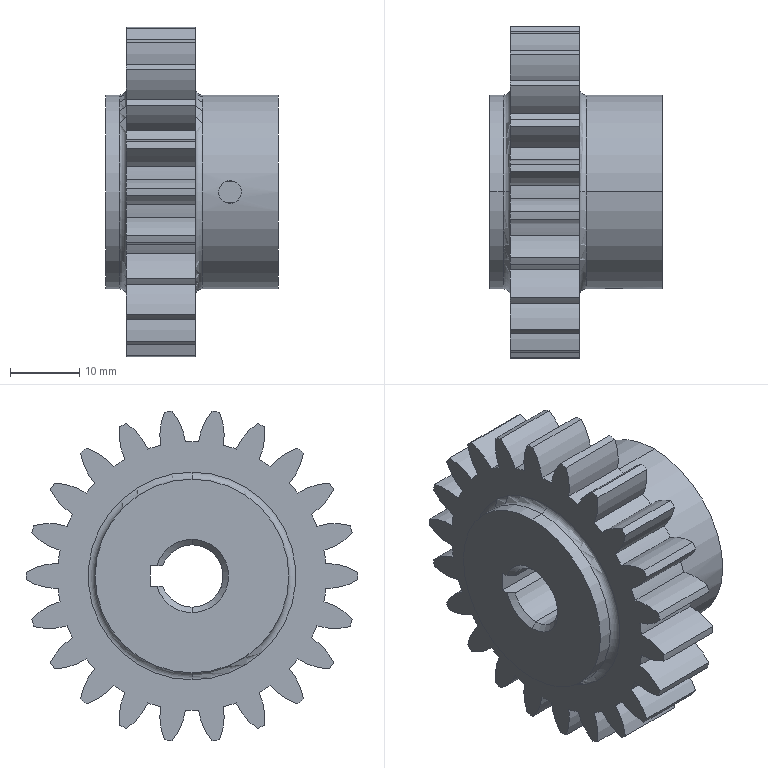Component | SolidWorks | AxisGear(Modified)-1 | 1 solid | 116 faces | box 25 x 47.98 x 47.63 mm | volume 22179 mm3 | cylinder 102 | plane 7 | torus 4 | cone 3 | commonest cylinder face diameters 17.6 x48 38.857 x23 47.978 x22 28 x4 9 x3 3.3 x2 | material AISI 1045 Steel, Cold Drawn
build123d program:
from build123d import *

# Parameters (mm, degrees)
SKETCH1_R                     = 14
BOSS_EXTRUDE1_DEPTH           = 10
BOSS_EXTRUDE2_DEPTH           = 22
BOSS_EXTRUDE2_DEPTH_BACK      = 3
SKETCH2_R                     = 14
M4_TAPPED_HOLE_DRILL_2_REACH  = 52.709
M4_TAPPED_HOLE_DRILL_2_BORE_R = 1.65
FILLET1_R                     = 1
CHAMFER1_SIZE                 = 0.8


with BuildPart() as part:
    # Sketch1 → Boss-Extrude1 (new body)
    with BuildSketch(Plane.XY):
        with BuildLine():
            ThreePointArc((-11.984, 15.293), (-12.723, 14.683), (-13.432, 14.038))
            ThreePointArc((-13.432, 14.038), (-15.452, 15.382), (-17.762, 16.124))
            ThreePointArc((-17.762, 16.124), (-18.13, 15.709), (-18.488, 15.287))
            ThreePointArc((-18.488, 15.287), (-17.425, 13.105), (-15.807, 11.297))
            ThreePointArc((-15.807, 11.297), (-16.344, 10.504), (-16.842, 9.685))
            ThreePointArc((-16.842, 9.685), (-19.159, 10.406), (-21.585, 10.467))
            ThreePointArc((-21.585, 10.467), (-21.821, 9.965), (-22.045, 9.459))
            ThreePointArc((-22.045, 9.459), (-20.411, 7.665), (-18.349, 6.386))
            ThreePointArc((-18.349, 6.386), (-18.642, 5.474), (-18.889, 4.548))
            ThreePointArc((-18.889, 4.548), (-21.315, 4.587), (-23.66, 3.961))
            ThreePointArc((-23.66, 3.961), (-23.745, 3.414), (-23.817, 2.865))
            ThreePointArc((-23.817, 2.865), (-21.744, 1.604), (-19.405, 0.9579))
            ThreePointArc((-19.405, 0.9579), (-19.429, 0), (-19.405, -0.9579))
            ThreePointArc((-19.405, -0.9579), (-21.744, -1.604), (-23.817, -2.865))
            ThreePointArc((-23.817, -2.865), (-23.745, -3.414), (-23.66, -3.961))
            ThreePointArc((-23.66, -3.961), (-21.315, -4.587), (-18.889, -4.548))
            ThreePointArc((-18.889, -4.548), (-18.642, -5.474), (-18.349, -6.386))
            ThreePointArc((-18.349, -6.386), (-20.411, -7.665), (-22.045, -9.459))
            ThreePointArc((-22.045, -9.459), (-21.821, -9.965), (-21.585, -10.467))
            ThreePointArc((-21.585, -10.467), (-19.159, -10.406), (-16.842, -9.685))
            ThreePointArc((-16.842, -9.685), (-16.344, -10.504), (-15.807, -11.297))
            ThreePointArc((-15.807, -11.297), (-17.425, -13.105), (-18.488, -15.287))
            ThreePointArc((-18.488, -15.287), (-18.13, -15.709), (-17.762, -16.124))
            ThreePointArc((-17.762, -16.124), (-15.452, -15.382), (-13.432, -14.038))
            ThreePointArc((-13.432, -14.038), (-12.723, -14.683), (-11.984, -15.293))
            ThreePointArc((-11.984, -15.293), (-13.027, -17.483), (-13.432, -19.876))
            ThreePointArc((-13.432, -19.876), (-12.969, -20.181), (-12.5, -20.475))
            ThreePointArc((-12.5, -20.475), (-10.492, -19.113), (-8.932, -17.254))
            ThreePointArc((-8.932, -17.254), (-8.071, -17.673), (-7.19, -18.049))
            ThreePointArc((-7.19, -18.049), (-7.573, -20.445), (-7.288, -22.855))
            ThreePointArc((-7.288, -22.855), (-6.758, -23.017), (-6.225, -23.167))
            ThreePointArc((-6.225, -23.167), (-4.682, -21.294), (-3.71, -19.071))
            ThreePointArc((-3.71, -19.071), (-2.765, -19.231), (-1.813, -19.344))
            ThreePointArc((-1.813, -19.344), (-1.507, -21.751), (-0.554, -23.983))
            ThreePointArc((-0.554, -23.983), (0, -23.989), (0.554, -23.983))
            ThreePointArc((0.554, -23.983), (1.507, -21.751), (1.813, -19.344))
            ThreePointArc((1.813, -19.344), (2.765, -19.231), (3.71, -19.071))
            ThreePointArc((3.71, -19.071), (4.682, -21.294), (6.225, -23.167))
            ThreePointArc((6.225, -23.167), (6.758, -23.017), (7.288, -22.855))
            ThreePointArc((7.288, -22.855), (7.573, -20.445), (7.19, -18.049))
            ThreePointArc((7.19, -18.049), (8.071, -17.673), (8.932, -17.254))
            ThreePointArc((8.932, -17.254), (10.492, -19.113), (12.5, -20.475))
            ThreePointArc((12.5, -20.475), (12.969, -20.181), (13.432, -19.876))
            ThreePointArc((13.432, -19.876), (13.027, -17.483), (11.984, -15.293))
            ThreePointArc((11.984, -15.293), (12.723, -14.683), (13.432, -14.038))
            ThreePointArc((13.432, -14.038), (15.452, -15.382), (17.762, -16.124))
            ThreePointArc((17.762, -16.124), (18.13, -15.709), (18.488, -15.287))
            ThreePointArc((18.488, -15.287), (17.425, -13.105), (15.807, -11.297))
            ThreePointArc((15.807, -11.297), (16.344, -10.504), (16.842, -9.685))
            ThreePointArc((16.842, -9.685), (19.159, -10.406), (21.585, -10.467))
            ThreePointArc((21.585, -10.467), (21.821, -9.965), (22.045, -9.459))
            ThreePointArc((22.045, -9.459), (20.411, -7.665), (18.349, -6.386))
            ThreePointArc((18.349, -6.386), (18.642, -5.474), (18.889, -4.548))
            ThreePointArc((18.889, -4.548), (21.315, -4.587), (23.66, -3.961))
            ThreePointArc((23.66, -3.961), (23.745, -3.414), (23.817, -2.865))
            ThreePointArc((23.817, -2.865), (21.744, -1.604), (19.405, -0.9579))
            ThreePointArc((19.405, -0.9579), (19.429, 0), (19.405, 0.9579))
            ThreePointArc((19.405, 0.9579), (21.744, 1.604), (23.817, 2.865))
            ThreePointArc((23.817, 2.865), (23.745, 3.414), (23.66, 3.961))
            ThreePointArc((23.66, 3.961), (21.315, 4.587), (18.889, 4.548))
            ThreePointArc((18.889, 4.548), (18.642, 5.474), (18.349, 6.386))
            ThreePointArc((18.349, 6.386), (20.411, 7.665), (22.045, 9.459))
            ThreePointArc((22.045, 9.459), (21.821, 9.965), (21.585, 10.467))
            ThreePointArc((21.585, 10.467), (19.159, 10.406), (16.842, 9.685))
            ThreePointArc((16.842, 9.685), (16.344, 10.504), (15.807, 11.297))
            ThreePointArc((15.807, 11.297), (17.425, 13.105), (18.488, 15.287))
            ThreePointArc((18.488, 15.287), (18.13, 15.709), (17.762, 16.124))
            ThreePointArc((17.762, 16.124), (15.452, 15.382), (13.432, 14.038))
            ThreePointArc((13.432, 14.038), (12.723, 14.683), (11.984, 15.293))
            ThreePointArc((11.984, 15.293), (13.027, 17.483), (13.432, 19.876))
            ThreePointArc((13.432, 19.876), (12.969, 20.181), (12.5, 20.475))
            ThreePointArc((12.5, 20.475), (10.492, 19.113), (8.932, 17.254))
            ThreePointArc((8.932, 17.254), (8.071, 17.673), (7.19, 18.049))
            ThreePointArc((7.19, 18.049), (7.573, 20.445), (7.288, 22.855))
            ThreePointArc((7.288, 22.855), (6.758, 23.017), (6.225, 23.167))
            ThreePointArc((6.225, 23.167), (4.682, 21.294), (3.71, 19.071))
            ThreePointArc((3.71, 19.071), (2.765, 19.231), (1.813, 19.344))
            ThreePointArc((1.813, 19.344), (1.507, 21.751), (0.554, 23.983))
            ThreePointArc((0.554, 23.983), (0, 23.989), (-0.554, 23.983))
            ThreePointArc((-0.554, 23.983), (-1.507, 21.751), (-1.813, 19.344))
            ThreePointArc((-1.813, 19.344), (-2.765, 19.231), (-3.71, 19.071))
            ThreePointArc((-3.71, 19.071), (-4.682, 21.294), (-6.225, 23.167))
            ThreePointArc((-6.225, 23.167), (-6.758, 23.017), (-7.288, 22.855))
            ThreePointArc((-7.288, 22.855), (-7.573, 20.445), (-7.19, 18.049))
            ThreePointArc((-7.19, 18.049), (-8.071, 17.673), (-8.932, 17.254))
            ThreePointArc((-8.932, 17.254), (-10.492, 19.113), (-12.5, 20.475))
            ThreePointArc((-12.5, 20.475), (-12.969, 20.181), (-13.432, 19.876))
            ThreePointArc((-13.432, 19.876), (-13.027, 17.483), (-11.984, 15.293))
        make_face()
        Circle(SKETCH1_R, mode=Mode.SUBTRACT)
    extrude(amount=BOSS_EXTRUDE1_DEPTH)

    # Sketch2 → Boss-Extrude2 (add, two sides: drawn at the far end of the back side and taken through both)
    with BuildSketch(Plane.XY.offset(-BOSS_EXTRUDE2_DEPTH_BACK)):
        Circle(SKETCH2_R)
        with BuildLine():
            Line((-1.5, -6), (-1.5, -4.243))
            ThreePointArc((-1.5, -4.243), (0, 4.5), (1.5, -4.243))
            Line((1.5, -4.243), (1.5, -6))
            Line((1.5, -6), (-1.5, -6))
        make_face(mode=Mode.SUBTRACT)
    extrude(amount=BOSS_EXTRUDE2_DEPTH + BOSS_EXTRUDE2_DEPTH_BACK)

    # M4 Tapped Hole Drill 2 bore → M4 Tapped Hole Drill 2 (cut, up to next)
    with BuildSketch(Plane(origin=(0, 15, 0), x_dir=(1, 0, 0), z_dir=(0, 1, 0)), mode=Mode.PRIVATE) as m4_tapped_hole_drill_2_sk1:
        with Locations((0, -15)):
            Circle(M4_TAPPED_HOLE_DRILL_2_BORE_R)
    m4_tapped_hole_drill_2_tool1 = extrude(m4_tapped_hole_drill_2_sk1.sketch, amount=-M4_TAPPED_HOLE_DRILL_2_REACH, mode=Mode.PRIVATE) & part.part
    add(m4_tapped_hole_drill_2_tool1.solids().sort_by_distance((0, 15, 15))[0], mode=Mode.SUBTRACT)

    # Fillet1
    fillet1_edges = [part.edges().sort_by_distance(p)[0] for p in [
        (-14, 0, 10),
        (-14, 0, 0),
    ]]
    fillet(fillet1_edges, radius=FILLET1_R)

    # Chamfer1
    chamfer1_edges = [part.edges().sort_by_distance(p)[0] for p in [
        (0, 4.5, -3),
    ]]
    chamfer(chamfer1_edges, length=CHAMFER1_SIZE)


solid = part.part

# Placed as in the assembly
solid = solid.moved(Location((50.062, 15.116, 349), (180, 90, 0)))